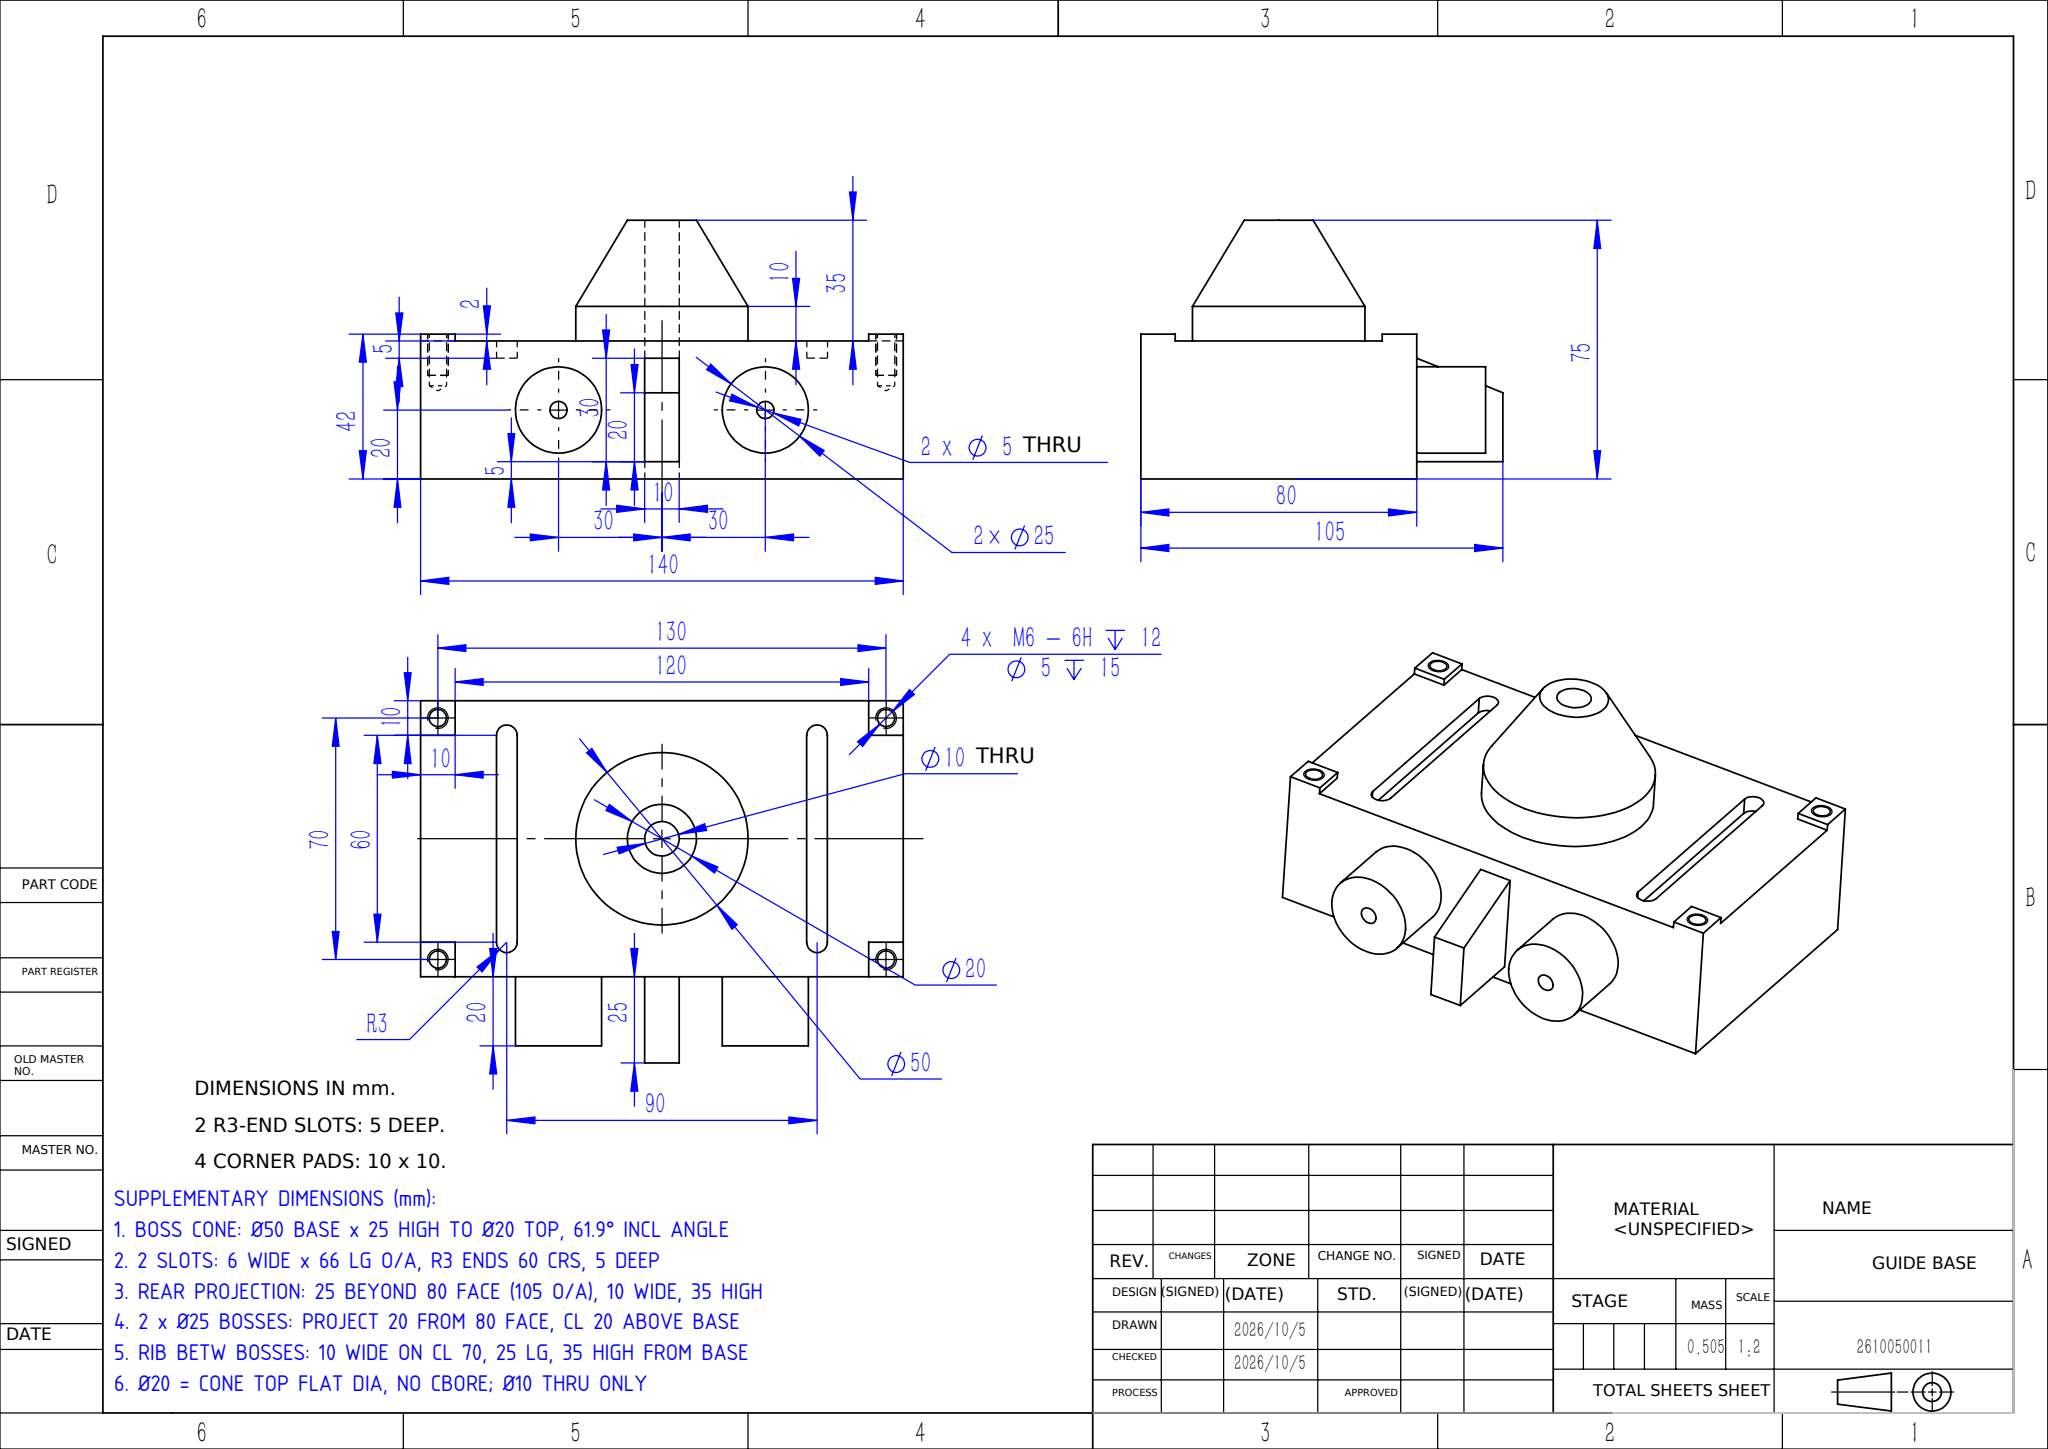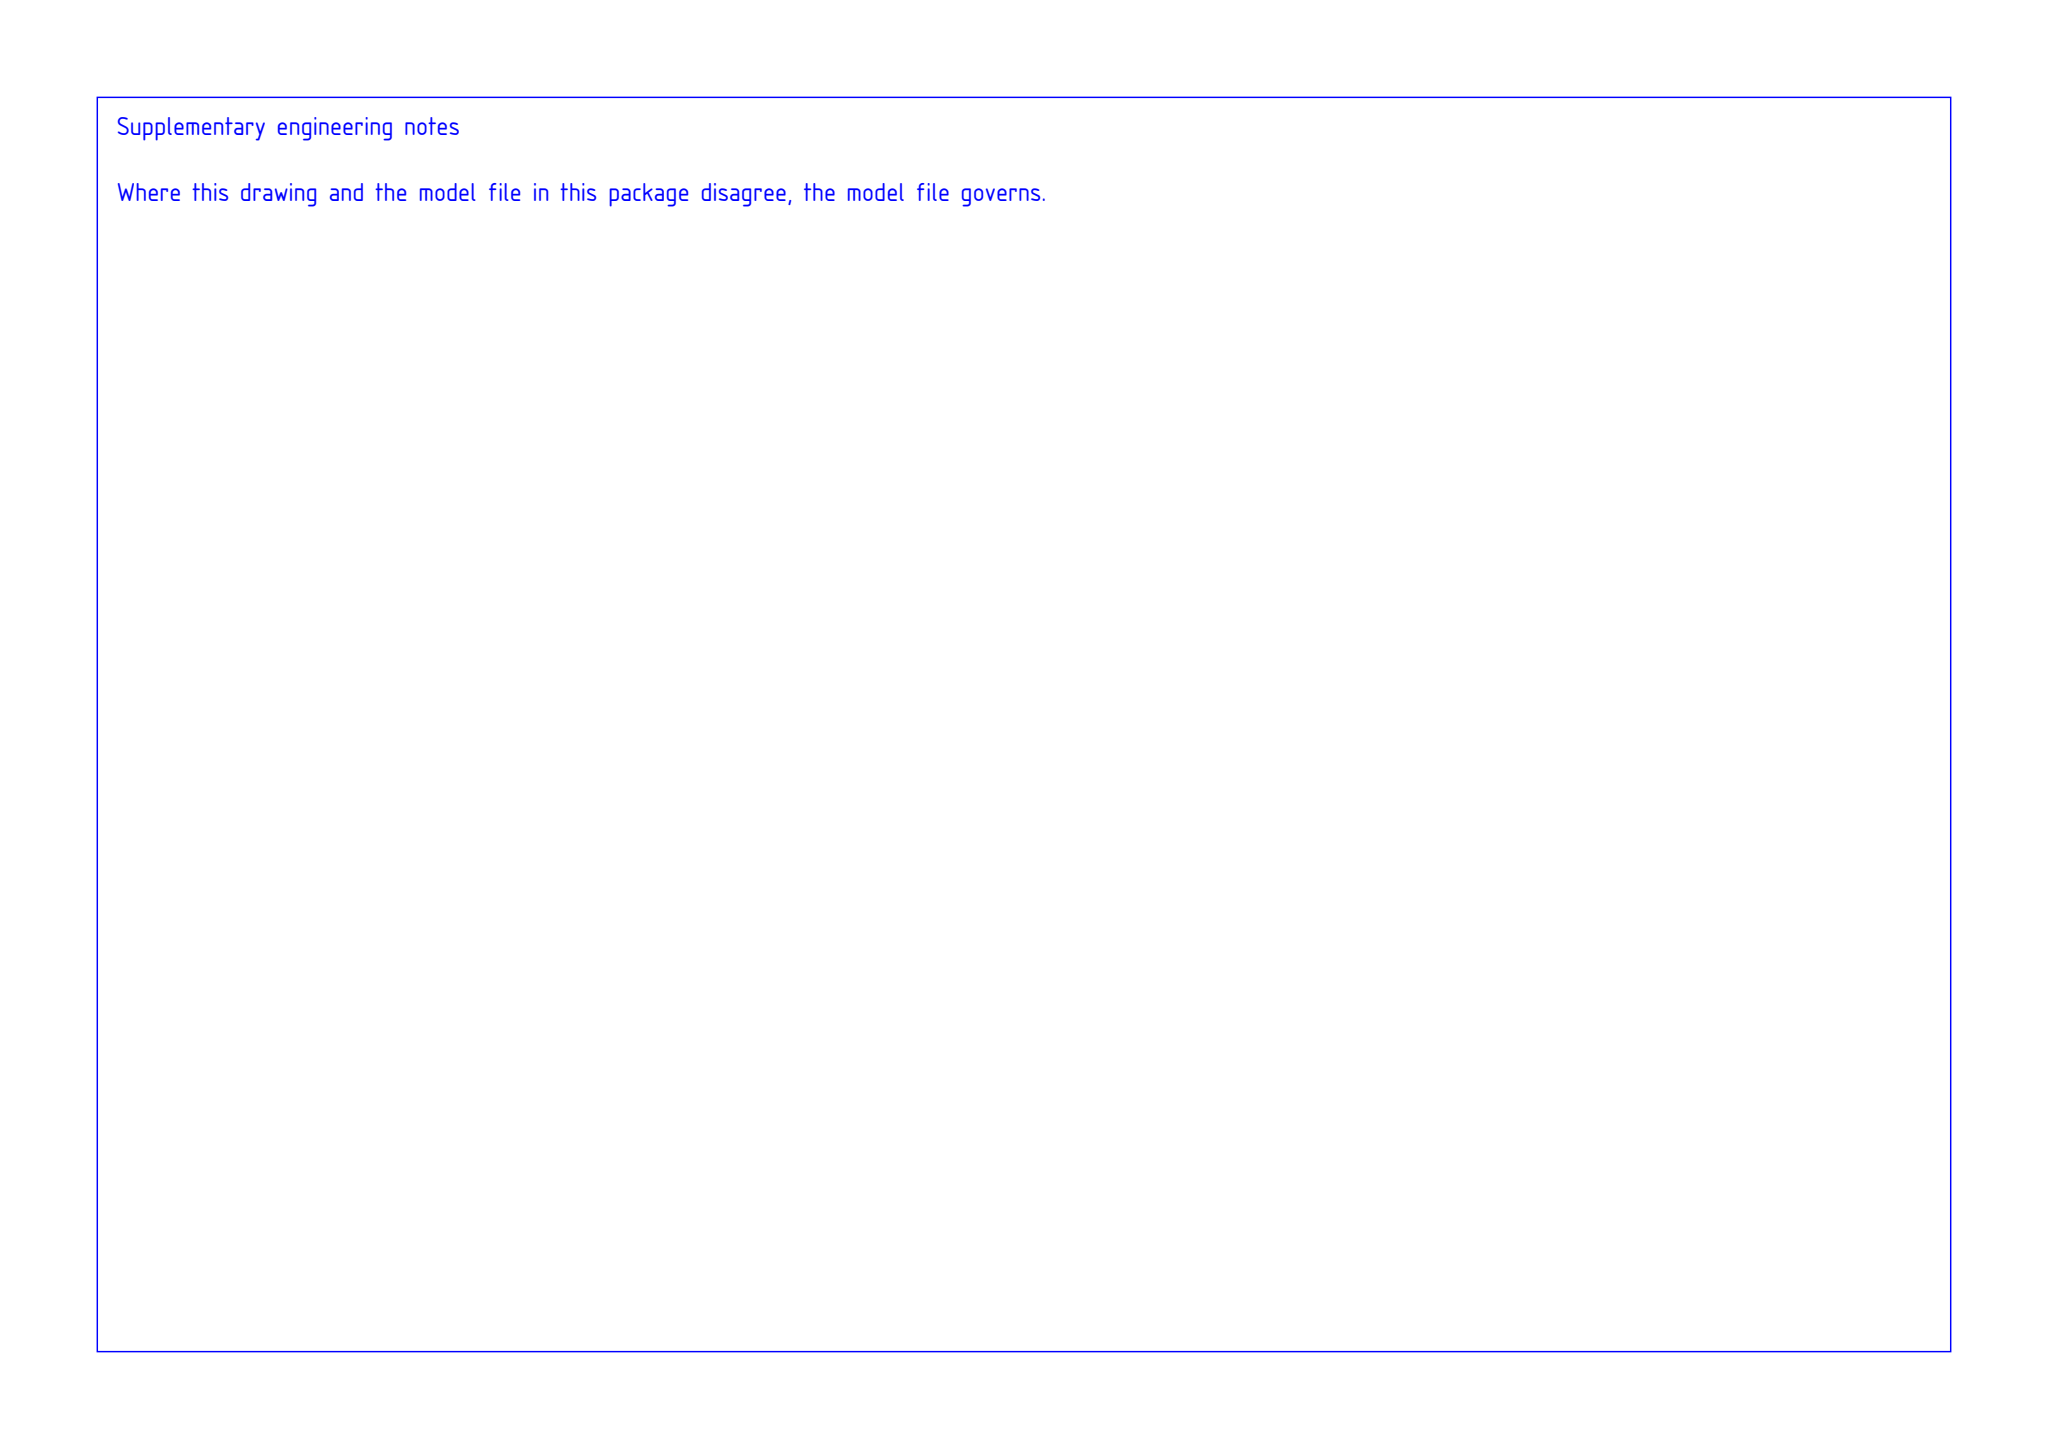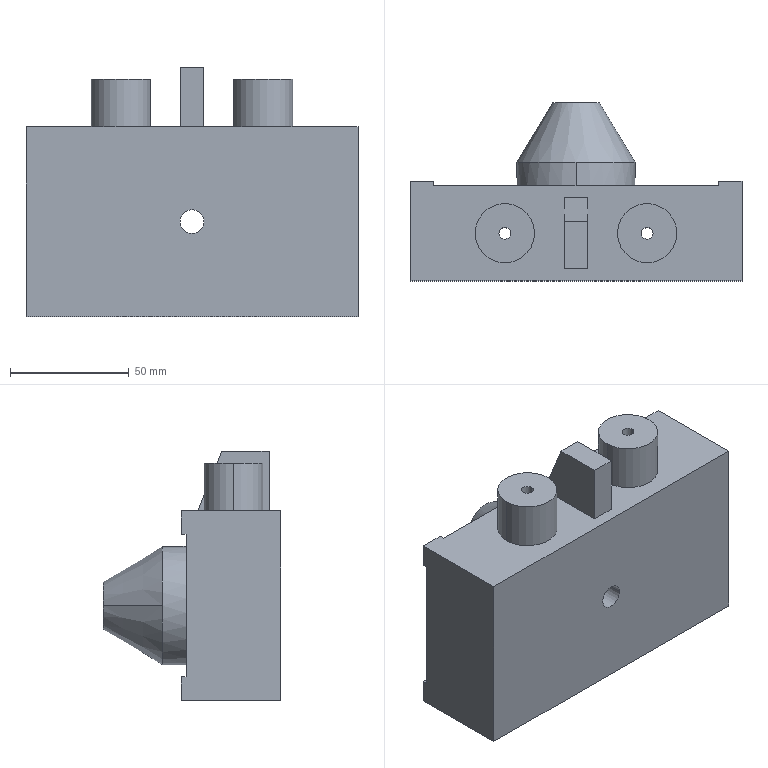Part | SolidWorks | mm | 1 solid | 68 faces | box 140 x 75 x 105 mm | volume 504928 mm3 | plane 32 | cylinder 26 | cone 10 | commonest cylinder face diameters 5 x12 6 x6 25 x4 10 x2 50 x2
build123d program:
from build123d import *

# Parameters (mm, degrees)
SKETCH1_W                = 140
SKETCH1_H                = 80
BOSS_EXTRUDE1_DEPTH      = 20
SKETCH2_R                = 12.5
BOSS_EXTRUDE2_DEPTH      = 20
BOSS_EXTRUDE3_DEPTH      = 5
F_5_0_5_DIAMETER_HOLE1_D = 5
SKETCH8_W                = 10
SKETCH8_H                = 10
BOSS_EXTRUDE4_DEPTH      = 2
M6_TAPPED_HOLE1_D        = 5
M6_TAPPED_HOLE1_DEPTH    = 15
M6_TAPPED_HOLE1_TIP      = 1.502
SKETCH12_R               = 25
BOSS_EXTRUDE5_DEPTH      = 10
CUT_EXTRUDE1_DEPTH       = 5
SKETCH15_R               = 5
CUT_EXTRUDE2_DEPTH       = 122.45


with BuildPart() as part:
    # Sketch1 → Boss-Extrude1 (new, symmetric)
    with BuildSketch(Plane(origin=(0, 0, 0), x_dir=(1, 0, 0), z_dir=(0, 1, 0))):
        Rectangle(SKETCH1_W, SKETCH1_H)
    extrude(amount=BOSS_EXTRUDE1_DEPTH, both=True)

    # Sketch2 → Boss-Extrude2 (add)
    with BuildSketch(Plane.XY.offset(40)):
        with Locations(Location((-30, 0, 0), (0, 0, 180))):
            Circle(SKETCH2_R)
        with Locations(Location((30, 0, 0), (0, 0, 180))):
            Circle(SKETCH2_R)
    extrude(amount=BOSS_EXTRUDE2_DEPTH)

    # Sketch3 → Boss-Extrude3 (add, symmetric)
    with BuildSketch(Plane(origin=(0, 0, 0), x_dir=(0, 0, -1), z_dir=(1, 0, 0))):
        Polygon((-40, 15), (-65, 5), (-65, -15), (-40, -15), align=None)
    extrude(amount=BOSS_EXTRUDE3_DEPTH, both=True)

    # 5.0 _5_ Diameter Hole1 (through all)
    with Locations(Plane.XY.offset(60)):
        with Locations((-30, 0), (30, 0)):
            Hole(F_5_0_5_DIAMETER_HOLE1_D / 2)

    # Sketch8 → Boss-Extrude4 (add, symmetric)
    with BuildSketch(Plane(origin=(0, 20, 0), x_dir=(1, 0, 0), z_dir=(0, 1, 0))):
        with Locations((-65, 35)):
            Rectangle(SKETCH8_W, SKETCH8_H)
        with Locations((-65, -35)):
            Rectangle(SKETCH8_W, SKETCH8_H)
        with Locations((65, -35)):
            Rectangle(SKETCH8_W, SKETCH8_H)
        with Locations((65, 35)):
            Rectangle(SKETCH8_W, SKETCH8_H)
    extrude(amount=BOSS_EXTRUDE4_DEPTH, both=True)

    # M6 Tapped Hole1
    with Locations(Plane(origin=(0, 22, 0), x_dir=(1, 0, 0), z_dir=(0, 1, 0))):
        with Locations((-65, 35), (-65, -35), (65, -35), (65, 35)):
            Hole(M6_TAPPED_HOLE1_D / 2, depth=M6_TAPPED_HOLE1_DEPTH)
            with Locations((0, 0, -(M6_TAPPED_HOLE1_DEPTH + M6_TAPPED_HOLE1_TIP / 2))):  # 118° drill point
                Cone(0, M6_TAPPED_HOLE1_D / 2, M6_TAPPED_HOLE1_TIP, mode=Mode.SUBTRACT)

    # Sketch12 → Boss-Extrude5 (add, symmetric)
    with BuildSketch(Plane(origin=(0, 20, 0), x_dir=(1, 0, 0), z_dir=(0, 1, 0))):
        with Locations(Location((0, 0, 0), (0, 0, 90))):
            Circle(SKETCH12_R)
    extrude(amount=BOSS_EXTRUDE5_DEPTH, both=True)

    # Sketch13 → Revolve1 (revolve)
    with BuildSketch(Plane.XY, mode=Mode.PRIVATE) as revolve1_sk:
        Polygon((0, 30), (25, 30), (10, 55), (0, 55), align=None)
    revolve(revolve1_sk.sketch.rotate(Axis((0, 55, 0), (0, -1, 0)), 270), axis=Axis((0, 55, 0), (0, -1, 0)))

    # Sketch14 → Cut-Extrude1 (cut)
    with BuildSketch(Plane(origin=(0, 20, 0), x_dir=(1, 0, 0), z_dir=(0, 1, 0))):
        with BuildLine():
            Line((-42, 30), (-42, -30))
            ThreePointArc((-42, -30), (-45, -33), (-48, -30))
            Line((-48, -30), (-48, 30))
            ThreePointArc((-48, 30), (-45, 33), (-42, 30))
        make_face()
        with BuildLine():
            Line((42, 30), (42, -30))
            ThreePointArc((42, -30), (45, -33), (48, -30))
            Line((48, -30), (48, 30))
            ThreePointArc((48, 30), (45, 33), (42, 30))
        make_face()
    extrude(amount=-CUT_EXTRUDE1_DEPTH, mode=Mode.SUBTRACT)

    # Sketch15 → Cut-Extrude2 (cut, through all)
    with BuildSketch(Plane(origin=(0, 55, 0), x_dir=(1, 0, 0), z_dir=(0, 1, 0))):
        with Locations(Location((0, 0, 0), (0, 0, 180))):
            Circle(SKETCH15_R)
    extrude(amount=-CUT_EXTRUDE2_DEPTH, mode=Mode.SUBTRACT)


solid = part.part